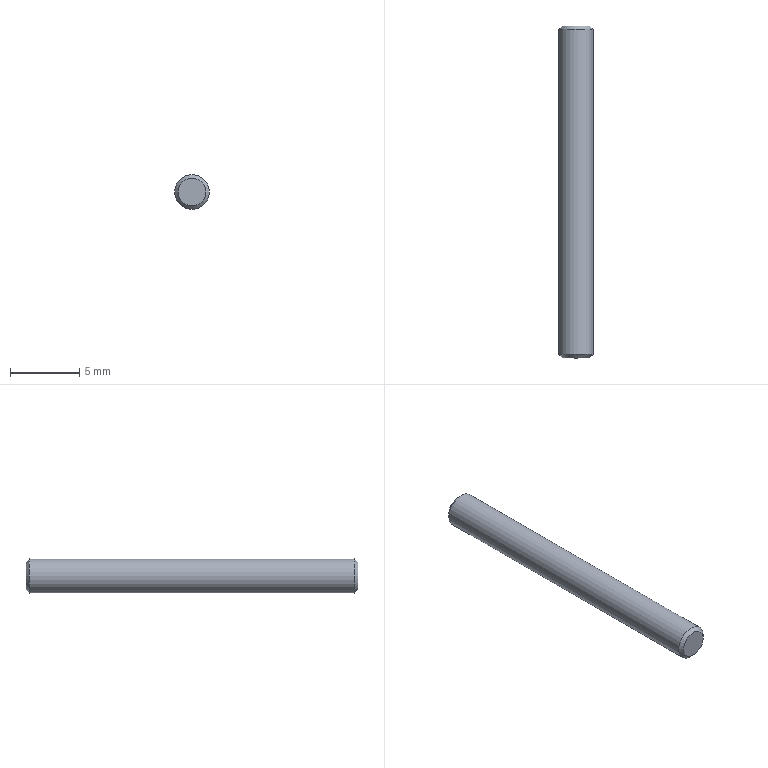Component | NX | CONNECTOR_2 | 1 solid | 5 faces | box 2.5 x 24 x 2.5 mm | volume 117 mm3 | plane 2 | cone 2 | cylinder 1 | commonest cylinder face diameters 2.5 x1
STEP:
#1=CARTESIAN_POINT('',(0.,0.,0.));
#2=DIRECTION('',(0.,0.,1.));
#3=DIRECTION('',(1.,0.,0.));
#4=AXIS2_PLACEMENT_3D('',#1,#2,#3);
#5=CARTESIAN_POINT('',(18.,12.,132.75));
#6=VERTEX_POINT('',#5);
#7=CARTESIAN_POINT('',(17.,12.,132.75));
#8=DIRECTION('',(0.,1.,0.));
#9=DIRECTION('',(1.,0.,0.));
#10=AXIS2_PLACEMENT_3D('',#7,#8,#9);
#11=CIRCLE('',#10,1.);
#12=CARTESIAN_POINT('',(17.,12.,132.75));
#13=DIRECTION('',(0.,1.,0.));
#14=DIRECTION('',(1.,0.,0.));
#15=AXIS2_PLACEMENT_3D('',#12,#13,#14);
#16=PLANE('',#15);
#17=CARTESIAN_POINT('',(0.,0.));
#18=DIRECTION('',(1.,0.));
#19=AXIS2_PLACEMENT_2D('',#17,#18);
#20=CIRCLE('',#19,1.);
#21=(GEOMETRIC_REPRESENTATION_CONTEXT(2)PARAMETRIC_REPRESENTATION_CONTEXT()REPRESENTATION_CONTEXT('',''));
#22=DEFINITIONAL_REPRESENTATION('',(#20),#21);
#23=PCURVE('',#16,#22);
#24=CARTESIAN_POINT('',(17.,11.75,132.75));
#25=DIRECTION('',(0.,-1.,0.));
#26=DIRECTION('',(-1.,0.,0.));
#27=AXIS2_PLACEMENT_3D('',#24,#25,#26);
#28=CONICAL_SURFACE('',#27,1.25,0.7854);
#29=CARTESIAN_POINT('',(9.425,-0.25));
#30=DIRECTION('',(-1.,0.));
#31=VECTOR('',#30,1.);
#32=LINE('',#29,#31);
#33=(GEOMETRIC_REPRESENTATION_CONTEXT(2)PARAMETRIC_REPRESENTATION_CONTEXT()REPRESENTATION_CONTEXT('',''));
#34=DEFINITIONAL_REPRESENTATION('',(#32),#33);
#35=PCURVE('',#28,#34);
#36=SURFACE_CURVE('',#11,(#23,#35),.PCURVE_S1.);
#37=EDGE_CURVE('',#6,#6,#36,.T.);
#38=ORIENTED_EDGE('',*,*,#37,.T.);
#39=EDGE_LOOP('',(#38));
#40=FACE_BOUND('',#39,.T.);
#41=ADVANCED_FACE('',(#40),#16,.T.);
#42=CARTESIAN_POINT('',(16.,-12.,132.75));
#43=VERTEX_POINT('',#42);
#44=CARTESIAN_POINT('',(17.,-12.,132.75));
#45=DIRECTION('',(0.,-1.,0.));
#46=DIRECTION('',(-1.,0.,0.));
#47=AXIS2_PLACEMENT_3D('',#44,#45,#46);
#48=CIRCLE('',#47,1.);
#49=CARTESIAN_POINT('',(17.,-12.,132.75));
#50=DIRECTION('',(0.,-1.,0.));
#51=DIRECTION('',(-1.,0.,0.));
#52=AXIS2_PLACEMENT_3D('',#49,#50,#51);
#53=PLANE('',#52);
#54=CARTESIAN_POINT('',(0.,0.));
#55=DIRECTION('',(1.,0.));
#56=AXIS2_PLACEMENT_2D('',#54,#55);
#57=CIRCLE('',#56,1.);
#58=(GEOMETRIC_REPRESENTATION_CONTEXT(2)PARAMETRIC_REPRESENTATION_CONTEXT()REPRESENTATION_CONTEXT('',''));
#59=DEFINITIONAL_REPRESENTATION('',(#57),#58);
#60=PCURVE('',#53,#59);
#61=CARTESIAN_POINT('',(17.,-11.75,132.75));
#62=DIRECTION('',(0.,1.,0.));
#63=DIRECTION('',(1.,0.,0.));
#64=AXIS2_PLACEMENT_3D('',#61,#62,#63);
#65=CONICAL_SURFACE('',#64,1.25,0.7854);
#66=CARTESIAN_POINT('',(9.425,-0.25));
#67=DIRECTION('',(-1.,0.));
#68=VECTOR('',#67,1.);
#69=LINE('',#66,#68);
#70=(GEOMETRIC_REPRESENTATION_CONTEXT(2)PARAMETRIC_REPRESENTATION_CONTEXT()REPRESENTATION_CONTEXT('',''));
#71=DEFINITIONAL_REPRESENTATION('',(#69),#70);
#72=PCURVE('',#65,#71);
#73=SURFACE_CURVE('',#48,(#60,#72),.PCURVE_S1.);
#74=EDGE_CURVE('',#43,#43,#73,.T.);
#75=ORIENTED_EDGE('',*,*,#74,.T.);
#76=EDGE_LOOP('',(#75));
#77=FACE_BOUND('',#76,.T.);
#78=ADVANCED_FACE('',(#77),#53,.T.);
#79=CARTESIAN_POINT('',(15.75,-11.75,132.75));
#80=VERTEX_POINT('',#79);
#81=CARTESIAN_POINT('',(18.25,-11.75,132.75));
#82=VERTEX_POINT('',#81);
#83=CARTESIAN_POINT('',(17.,-11.75,132.75));
#84=DIRECTION('',(0.,1.,0.));
#85=DIRECTION('',(-1.,0.,0.));
#86=AXIS2_PLACEMENT_3D('',#83,#84,#85);
#87=CIRCLE('',#86,1.25);
#88=CARTESIAN_POINT('',(17.,-12.,132.75));
#89=DIRECTION('',(0.,1.,0.));
#90=DIRECTION('',(1.,0.,0.));
#91=AXIS2_PLACEMENT_3D('',#88,#89,#90);
#92=CYLINDRICAL_SURFACE('',#91,1.25);
#93=CARTESIAN_POINT('',(3.142,0.25));
#94=DIRECTION('',(1.,0.));
#95=VECTOR('',#94,1.);
#96=LINE('',#93,#95);
#97=(GEOMETRIC_REPRESENTATION_CONTEXT(2)PARAMETRIC_REPRESENTATION_CONTEXT()REPRESENTATION_CONTEXT('',''));
#98=DEFINITIONAL_REPRESENTATION('',(#96),#97);
#99=PCURVE('',#92,#98);
#100=CARTESIAN_POINT('',(3.142,0.));
#101=DIRECTION('',(1.,0.));
#102=VECTOR('',#101,1.);
#103=LINE('',#100,#102);
#104=(GEOMETRIC_REPRESENTATION_CONTEXT(2)PARAMETRIC_REPRESENTATION_CONTEXT()REPRESENTATION_CONTEXT('',''));
#105=DEFINITIONAL_REPRESENTATION('',(#103),#104);
#106=PCURVE('',#65,#105);
#107=SURFACE_CURVE('',#87,(#99,#106),.PCURVE_S1.);
#108=EDGE_CURVE('',#80,#82,#107,.T.);
#109=ORIENTED_EDGE('',*,*,#108,.T.);
#110=CARTESIAN_POINT('',(18.25,11.75,132.75));
#111=VERTEX_POINT('',#110);
#112=CARTESIAN_POINT('',(18.25,-11.75,132.75));
#113=CARTESIAN_POINT('',(18.25,11.75,132.75));
#114=B_SPLINE_CURVE_WITH_KNOTS('',1,(#112,#113),.UNSPECIFIED.,.F.,.F.,(2,2),(0.25,23.75),.PIECEWISE_BEZIER_KNOTS.);
#115=CARTESIAN_POINT('',(6.283,0.));
#116=DIRECTION('',(0.,1.));
#117=VECTOR('',#116,1.);
#118=LINE('',#115,#117);
#119=(GEOMETRIC_REPRESENTATION_CONTEXT(2)PARAMETRIC_REPRESENTATION_CONTEXT()REPRESENTATION_CONTEXT('',''));
#120=DEFINITIONAL_REPRESENTATION('',(#118),#119);
#121=PCURVE('',#92,#120);
#122=CARTESIAN_POINT('',(0.,0.));
#123=DIRECTION('',(0.,1.));
#124=VECTOR('',#123,1.);
#125=LINE('',#122,#124);
#126=(GEOMETRIC_REPRESENTATION_CONTEXT(2)PARAMETRIC_REPRESENTATION_CONTEXT()REPRESENTATION_CONTEXT('',''));
#127=DEFINITIONAL_REPRESENTATION('',(#125),#126);
#128=PCURVE('',#92,#127);
#129=SEAM_CURVE('',#114,(#121,#128),.PCURVE_S1.);
#130=EDGE_CURVE('',#82,#111,#129,.T.);
#131=ORIENTED_EDGE('',*,*,#130,.T.);
#132=CARTESIAN_POINT('',(17.,11.75,132.75));
#133=DIRECTION('',(0.,-1.,0.));
#134=DIRECTION('',(1.,0.,0.));
#135=AXIS2_PLACEMENT_3D('',#132,#133,#134);
#136=CIRCLE('',#135,1.25);
#137=CARTESIAN_POINT('',(6.283,23.75));
#138=DIRECTION('',(-1.,0.));
#139=VECTOR('',#138,1.);
#140=LINE('',#137,#139);
#141=(GEOMETRIC_REPRESENTATION_CONTEXT(2)PARAMETRIC_REPRESENTATION_CONTEXT()REPRESENTATION_CONTEXT('',''));
#142=DEFINITIONAL_REPRESENTATION('',(#140),#141);
#143=PCURVE('',#92,#142);
#144=CARTESIAN_POINT('',(3.142,0.));
#145=DIRECTION('',(1.,0.));
#146=VECTOR('',#145,1.);
#147=LINE('',#144,#146);
#148=(GEOMETRIC_REPRESENTATION_CONTEXT(2)PARAMETRIC_REPRESENTATION_CONTEXT()REPRESENTATION_CONTEXT('',''));
#149=DEFINITIONAL_REPRESENTATION('',(#147),#148);
#150=PCURVE('',#28,#149);
#151=SURFACE_CURVE('',#136,(#143,#150),.PCURVE_S1.);
#152=EDGE_CURVE('',#111,#111,#151,.T.);
#153=ORIENTED_EDGE('',*,*,#152,.T.);
#154=ORIENTED_EDGE('',*,*,#130,.F.);
#155=CARTESIAN_POINT('',(17.,-11.75,132.75));
#156=DIRECTION('',(0.,1.,0.));
#157=DIRECTION('',(-1.,0.,0.));
#158=AXIS2_PLACEMENT_3D('',#155,#156,#157);
#159=CIRCLE('',#158,1.25);
#160=CARTESIAN_POINT('',(-3.142,0.25));
#161=DIRECTION('',(1.,0.));
#162=VECTOR('',#161,1.);
#163=LINE('',#160,#162);
#164=(GEOMETRIC_REPRESENTATION_CONTEXT(2)PARAMETRIC_REPRESENTATION_CONTEXT()REPRESENTATION_CONTEXT('',''));
#165=DEFINITIONAL_REPRESENTATION('',(#163),#164);
#166=PCURVE('',#92,#165);
#167=CARTESIAN_POINT('',(3.142,0.));
#168=DIRECTION('',(1.,0.));
#169=VECTOR('',#168,1.);
#170=LINE('',#167,#169);
#171=(GEOMETRIC_REPRESENTATION_CONTEXT(2)PARAMETRIC_REPRESENTATION_CONTEXT()REPRESENTATION_CONTEXT('',''));
#172=DEFINITIONAL_REPRESENTATION('',(#170),#171);
#173=PCURVE('',#65,#172);
#174=SURFACE_CURVE('',#159,(#166,#173),.PCURVE_S1.);
#175=EDGE_CURVE('',#82,#80,#174,.T.);
#176=ORIENTED_EDGE('',*,*,#175,.T.);
#177=EDGE_LOOP('',(#109,#131,#153,#154,#176));
#178=FACE_BOUND('',#177,.T.);
#179=ADVANCED_FACE('',(#178),#92,.T.);
#180=ORIENTED_EDGE('',*,*,#74,.F.);
#181=CARTESIAN_POINT('',(16.,-12.,132.75));
#182=CARTESIAN_POINT('',(15.75,-11.75,132.75));
#183=B_SPLINE_CURVE_WITH_KNOTS('',1,(#181,#182),.UNSPECIFIED.,.F.,.F.,(2,2),(-0.3536,0.),.PIECEWISE_BEZIER_KNOTS.);
#184=CARTESIAN_POINT('',(9.425,0.));
#185=DIRECTION('',(0.,1.));
#186=VECTOR('',#185,1.);
#187=LINE('',#184,#186);
#188=(GEOMETRIC_REPRESENTATION_CONTEXT(2)PARAMETRIC_REPRESENTATION_CONTEXT()REPRESENTATION_CONTEXT('',''));
#189=DEFINITIONAL_REPRESENTATION('',(#187),#188);
#190=PCURVE('',#65,#189);
#191=CARTESIAN_POINT('',(3.142,0.));
#192=DIRECTION('',(0.,1.));
#193=VECTOR('',#192,1.);
#194=LINE('',#191,#193);
#195=(GEOMETRIC_REPRESENTATION_CONTEXT(2)PARAMETRIC_REPRESENTATION_CONTEXT()REPRESENTATION_CONTEXT('',''));
#196=DEFINITIONAL_REPRESENTATION('',(#194),#195);
#197=PCURVE('',#65,#196);
#198=SEAM_CURVE('',#183,(#190,#197),.PCURVE_S1.);
#199=EDGE_CURVE('',#43,#80,#198,.T.);
#200=ORIENTED_EDGE('',*,*,#199,.T.);
#201=ORIENTED_EDGE('',*,*,#175,.F.);
#202=ORIENTED_EDGE('',*,*,#108,.F.);
#203=ORIENTED_EDGE('',*,*,#199,.F.);
#204=EDGE_LOOP('',(#180,#200,#201,#202,#203));
#205=FACE_BOUND('',#204,.T.);
#206=ADVANCED_FACE('',(#205),#65,.T.);
#207=ORIENTED_EDGE('',*,*,#37,.F.);
#208=CARTESIAN_POINT('',(18.,12.,132.75));
#209=CARTESIAN_POINT('',(18.25,11.75,132.75));
#210=B_SPLINE_CURVE_WITH_KNOTS('',1,(#208,#209),.UNSPECIFIED.,.F.,.F.,(2,2),(-0.3536,0.),.PIECEWISE_BEZIER_KNOTS.);
#211=CARTESIAN_POINT('',(9.425,0.));
#212=DIRECTION('',(0.,1.));
#213=VECTOR('',#212,1.);
#214=LINE('',#211,#213);
#215=(GEOMETRIC_REPRESENTATION_CONTEXT(2)PARAMETRIC_REPRESENTATION_CONTEXT()REPRESENTATION_CONTEXT('',''));
#216=DEFINITIONAL_REPRESENTATION('',(#214),#215);
#217=PCURVE('',#28,#216);
#218=CARTESIAN_POINT('',(3.142,0.));
#219=DIRECTION('',(0.,1.));
#220=VECTOR('',#219,1.);
#221=LINE('',#218,#220);
#222=(GEOMETRIC_REPRESENTATION_CONTEXT(2)PARAMETRIC_REPRESENTATION_CONTEXT()REPRESENTATION_CONTEXT('',''));
#223=DEFINITIONAL_REPRESENTATION('',(#221),#222);
#224=PCURVE('',#28,#223);
#225=SEAM_CURVE('',#210,(#217,#224),.PCURVE_S1.);
#226=EDGE_CURVE('',#6,#111,#225,.T.);
#227=ORIENTED_EDGE('',*,*,#226,.T.);
#228=ORIENTED_EDGE('',*,*,#152,.F.);
#229=ORIENTED_EDGE('',*,*,#226,.F.);
#230=EDGE_LOOP('',(#207,#227,#228,#229));
#231=FACE_BOUND('',#230,.T.);
#232=ADVANCED_FACE('',(#231),#28,.T.);
#233=CLOSED_SHELL('',(#41,#78,#179,#206,#232));
#234=MANIFOLD_SOLID_BREP('',#233);
#235=(LENGTH_UNIT()NAMED_UNIT(*)SI_UNIT(.MILLI.,.METRE.));
#236=UNCERTAINTY_MEASURE_WITH_UNIT(LENGTH_MEASURE(0.00001),#235,'','');
#237=(NAMED_UNIT(*)PLANE_ANGLE_UNIT()SI_UNIT($,.RADIAN.));
#238=(NAMED_UNIT(*)SI_UNIT($,.STERADIAN.)SOLID_ANGLE_UNIT());
#239=(GEOMETRIC_REPRESENTATION_CONTEXT(3)GLOBAL_UNCERTAINTY_ASSIGNED_CONTEXT((#236))GLOBAL_UNIT_ASSIGNED_CONTEXT((#235,#237,#238))REPRESENTATION_CONTEXT('',''));
#240=ADVANCED_BREP_SHAPE_REPRESENTATION('',(#4,#234),#239);